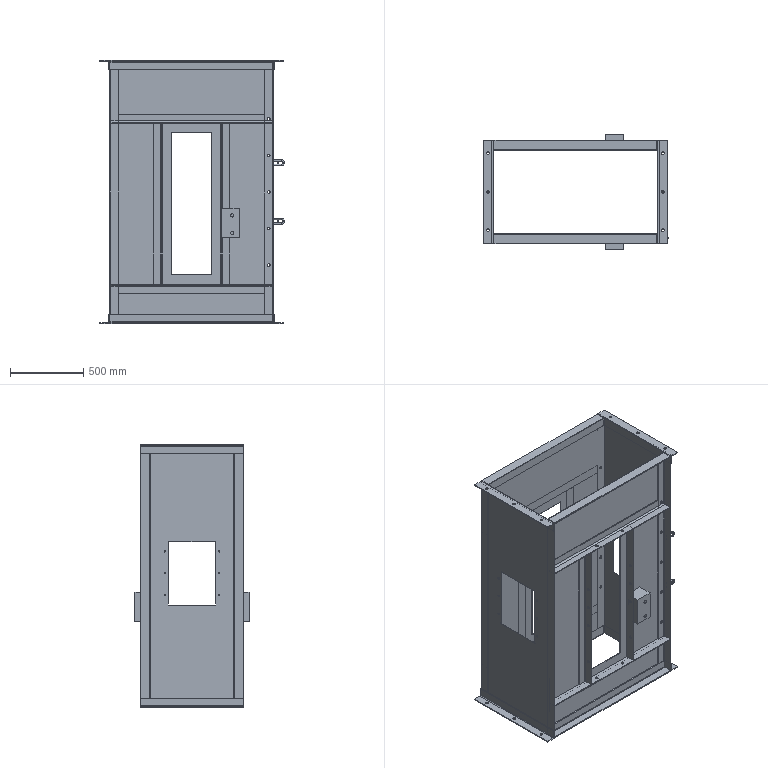Component | SolidWorks | LowerCasing-1 | 23 solids | 440 faces | volume 37623137 mm3 | plane 230 | cylinder 194 | torus 16 | commonest cylinder face diameters 18 x120 10 x28 12 x22 9 x12 22 x8 20 x4